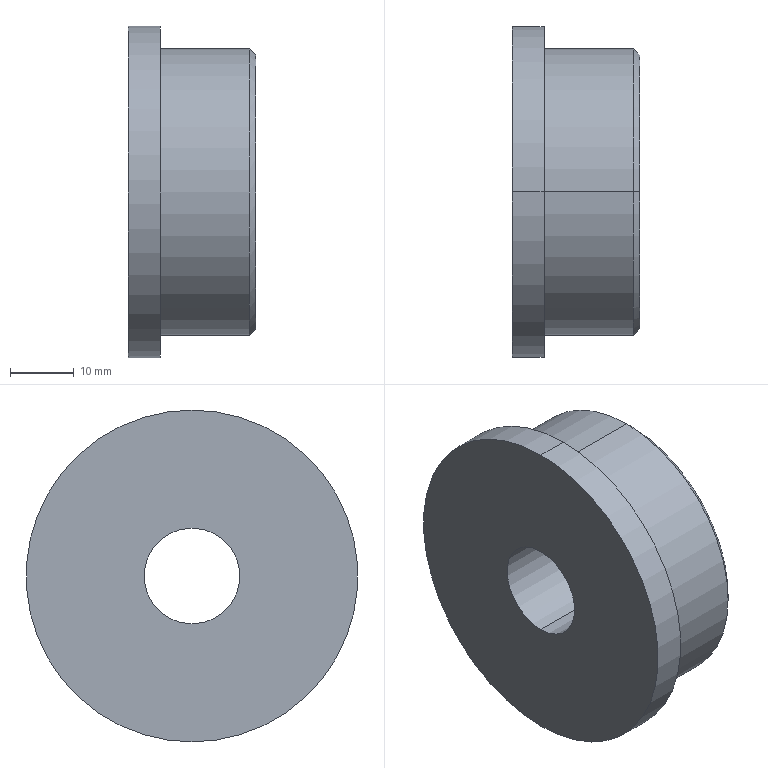Component | SolidWorks | GuideMechanism-1_RollerEndCap02-1 | 1 solid | 11 faces | box 20 x 52 x 52 mm | volume 30871 mm3 | cylinder 6 | plane 3 | cone 2 | commonest cylinder face diameters 52 x2 45 x2 15 x2
build123d program:
from build123d import *

# Parameters (mm, degrees)
CHAMFER1_SIZE = 1


with BuildPart() as part:
    # Sketch1 → Revolve1 (revolve)
    with BuildSketch(Plane.XY, mode=Mode.PRIVATE) as revolve1_sk:
        Polygon((7.5, 0), (7.5, 20), (22.5, 20), (22.5, 5), (26, 5), (26, 0), align=None)
    revolve(revolve1_sk.sketch.rotate(Axis((0, 0, 0), (0, 1, 0)), 90), axis=Axis((0, 0, 0), (0, 1, 0)))

    # Chamfer1
    chamfer1_edges = [part.edges().sort_by_distance(p)[0] for p in [
        (0, 20, 22.5),
    ]]
    chamfer(chamfer1_edges, length=CHAMFER1_SIZE)


solid = part.part

# Placed as in the assembly
solid = solid.moved(Location((-496.772, -352.564, 1209.912), (0, 0, -90)))
STEP:
#1=COLOUR_RGB('',0.7922,0.8196,0.9333);
#2=FILL_AREA_STYLE_COLOUR('',#1);
#3=FILL_AREA_STYLE('',(#2));
#4=SURFACE_STYLE_FILL_AREA(#3);
#5=SURFACE_SIDE_STYLE('',(#4));
#6=SURFACE_STYLE_USAGE(.BOTH.,#5);
#7=PRESENTATION_STYLE_ASSIGNMENT((#6));
#8=CARTESIAN_POINT('',(-18.771,-13.88,48.481));
#9=VERTEX_POINT('',#8);
#10=CARTESIAN_POINT('',(-18.771,-13.88,46.788));
#11=VERTEX_POINT('',#10);
#12=CARTESIAN_POINT('',(-18.771,-13.88,47.634));
#13=DIRECTION('',(1.,0.,0.));
#14=DIRECTION('',(0.,0.,1.));
#15=AXIS2_PLACEMENT_3D('',#12,#13,#14);
#16=CIRCLE('',#15,0.8465);
#17=EDGE_CURVE('',#9,#11,#16,.T.);
#18=ORIENTED_EDGE('',*,*,#17,.F.);
#19=CARTESIAN_POINT('',(-18.81,-13.88,48.52));
#20=VERTEX_POINT('',#19);
#21=CARTESIAN_POINT('',(-18.81,-13.88,48.52));
#22=DIRECTION('',(-0.7071,-0.,0.7071));
#23=VECTOR('',#22,39.37);
#24=LINE('',#21,#23);
#25=EDGE_CURVE('',#9,#20,#24,.T.);
#26=ORIENTED_EDGE('',*,*,#25,.T.);
#27=CARTESIAN_POINT('',(-18.81,-13.88,46.749));
#28=VERTEX_POINT('',#27);
#29=CARTESIAN_POINT('',(-18.81,-13.88,47.634));
#30=DIRECTION('',(-1.,-0.,-0.));
#31=DIRECTION('',(0.,0.,1.));
#32=AXIS2_PLACEMENT_3D('',#29,#30,#31);
#33=CIRCLE('',#32,0.8858);
#34=EDGE_CURVE('',#28,#20,#33,.T.);
#35=ORIENTED_EDGE('',*,*,#34,.F.);
#36=CARTESIAN_POINT('',(-18.81,-13.88,46.749));
#37=DIRECTION('',(-0.7071,0.,-0.7071));
#38=VECTOR('',#37,39.37);
#39=LINE('',#36,#38);
#40=EDGE_CURVE('',#11,#28,#39,.T.);
#41=ORIENTED_EDGE('',*,*,#40,.F.);
#42=EDGE_LOOP('',(#18,#26,#35,#41));
#43=FACE_OUTER_BOUND('',#42,.T.);
#44=CARTESIAN_POINT('',(-18.81,-13.88,47.634));
#45=DIRECTION('',(-1.,-0.,-0.));
#46=DIRECTION('',(0.,0.,-1.));
#47=AXIS2_PLACEMENT_3D('',#44,#45,#46);
#48=CONICAL_SURFACE('',#47,0.8858,0.7854);
#49=ADVANCED_FACE('',(#43),#48,.T.);
#50=CARTESIAN_POINT('',(-19.361,-13.88,46.611));
#51=VERTEX_POINT('',#50);
#52=CARTESIAN_POINT('',(-19.361,-13.88,48.658));
#53=VERTEX_POINT('',#52);
#54=CARTESIAN_POINT('',(-19.361,-13.88,47.634));
#55=DIRECTION('',(-1.,-0.,-0.));
#56=DIRECTION('',(0.,0.,-1.));
#57=AXIS2_PLACEMENT_3D('',#54,#55,#56);
#58=CIRCLE('',#57,1.024);
#59=EDGE_CURVE('',#51,#53,#58,.T.);
#60=ORIENTED_EDGE('',*,*,#59,.T.);
#61=CARTESIAN_POINT('',(-19.558,-13.88,48.658));
#62=VERTEX_POINT('',#61);
#63=CARTESIAN_POINT('',(-19.558,-13.88,48.658));
#64=DIRECTION('',(-1.,-0.,-0.));
#65=VECTOR('',#64,39.37);
#66=LINE('',#63,#65);
#67=EDGE_CURVE('',#53,#62,#66,.T.);
#68=ORIENTED_EDGE('',*,*,#67,.T.);
#69=CARTESIAN_POINT('',(-19.558,-13.88,46.611));
#70=VERTEX_POINT('',#69);
#71=CARTESIAN_POINT('',(-19.558,-13.88,47.634));
#72=DIRECTION('',(-1.,-0.,-0.));
#73=DIRECTION('',(0.,0.,-1.));
#74=AXIS2_PLACEMENT_3D('',#71,#72,#73);
#75=CIRCLE('',#74,1.024);
#76=EDGE_CURVE('',#70,#62,#75,.T.);
#77=ORIENTED_EDGE('',*,*,#76,.F.);
#78=CARTESIAN_POINT('',(-19.558,-13.88,46.611));
#79=DIRECTION('',(-1.,-0.,-0.));
#80=VECTOR('',#79,39.37);
#81=LINE('',#78,#80);
#82=EDGE_CURVE('',#51,#70,#81,.T.);
#83=ORIENTED_EDGE('',*,*,#82,.F.);
#84=EDGE_LOOP('',(#60,#68,#77,#83));
#85=FACE_OUTER_BOUND('',#84,.T.);
#86=CARTESIAN_POINT('',(-19.558,-13.88,47.634));
#87=DIRECTION('',(-1.,-0.,-0.));
#88=DIRECTION('',(0.,0.,-1.));
#89=AXIS2_PLACEMENT_3D('',#86,#87,#88);
#90=CYLINDRICAL_SURFACE('',#89,1.024);
#91=ADVANCED_FACE('',(#85),#90,.T.);
#92=ORIENTED_EDGE('',*,*,#34,.T.);
#93=CARTESIAN_POINT('',(-19.361,-13.88,48.52));
#94=VERTEX_POINT('',#93);
#95=CARTESIAN_POINT('',(-19.558,-13.88,48.52));
#96=DIRECTION('',(-1.,-0.,-0.));
#97=VECTOR('',#96,39.37);
#98=LINE('',#95,#97);
#99=EDGE_CURVE('',#20,#94,#98,.T.);
#100=ORIENTED_EDGE('',*,*,#99,.T.);
#101=CARTESIAN_POINT('',(-19.361,-13.88,46.749));
#102=VERTEX_POINT('',#101);
#103=CARTESIAN_POINT('',(-19.361,-13.88,47.634));
#104=DIRECTION('',(-1.,-0.,-0.));
#105=DIRECTION('',(0.,0.,-1.));
#106=AXIS2_PLACEMENT_3D('',#103,#104,#105);
#107=CIRCLE('',#106,0.8858);
#108=EDGE_CURVE('',#102,#94,#107,.T.);
#109=ORIENTED_EDGE('',*,*,#108,.F.);
#110=CARTESIAN_POINT('',(-19.558,-13.88,46.749));
#111=DIRECTION('',(-1.,-0.,-0.));
#112=VECTOR('',#111,39.37);
#113=LINE('',#110,#112);
#114=EDGE_CURVE('',#28,#102,#113,.T.);
#115=ORIENTED_EDGE('',*,*,#114,.F.);
#116=EDGE_LOOP('',(#92,#100,#109,#115));
#117=FACE_OUTER_BOUND('',#116,.T.);
#118=CARTESIAN_POINT('',(-19.558,-13.88,47.634));
#119=DIRECTION('',(-1.,-0.,-0.));
#120=DIRECTION('',(0.,0.,-1.));
#121=AXIS2_PLACEMENT_3D('',#118,#119,#120);
#122=CYLINDRICAL_SURFACE('',#121,0.8858);
#123=ADVANCED_FACE('',(#117),#122,.T.);
#124=CARTESIAN_POINT('',(-18.771,-13.88,47.93));
#125=VERTEX_POINT('',#124);
#126=CARTESIAN_POINT('',(-18.771,-13.88,47.339));
#127=VERTEX_POINT('',#126);
#128=CARTESIAN_POINT('',(-18.771,-13.88,47.634));
#129=DIRECTION('',(-1.,-0.,-0.));
#130=DIRECTION('',(0.,0.,-1.));
#131=AXIS2_PLACEMENT_3D('',#128,#129,#130);
#132=CIRCLE('',#131,0.2953);
#133=EDGE_CURVE('',#125,#127,#132,.T.);
#134=ORIENTED_EDGE('',*,*,#133,.F.);
#135=CARTESIAN_POINT('',(-19.558,-13.88,47.93));
#136=VERTEX_POINT('',#135);
#137=CARTESIAN_POINT('',(-19.558,-13.88,47.93));
#138=DIRECTION('',(-1.,-0.,-0.));
#139=VECTOR('',#138,39.37);
#140=LINE('',#137,#139);
#141=EDGE_CURVE('',#125,#136,#140,.T.);
#142=ORIENTED_EDGE('',*,*,#141,.T.);
#143=CARTESIAN_POINT('',(-19.558,-13.88,47.339));
#144=VERTEX_POINT('',#143);
#145=CARTESIAN_POINT('',(-19.558,-13.88,47.634));
#146=DIRECTION('',(-1.,-0.,-0.));
#147=DIRECTION('',(0.,0.,-1.));
#148=AXIS2_PLACEMENT_3D('',#145,#146,#147);
#149=CIRCLE('',#148,0.2953);
#150=EDGE_CURVE('',#136,#144,#149,.T.);
#151=ORIENTED_EDGE('',*,*,#150,.T.);
#152=CARTESIAN_POINT('',(-19.558,-13.88,47.339));
#153=DIRECTION('',(-1.,-0.,-0.));
#154=VECTOR('',#153,39.37);
#155=LINE('',#152,#154);
#156=EDGE_CURVE('',#127,#144,#155,.T.);
#157=ORIENTED_EDGE('',*,*,#156,.F.);
#158=EDGE_LOOP('',(#134,#142,#151,#157));
#159=FACE_OUTER_BOUND('',#158,.T.);
#160=CARTESIAN_POINT('',(-19.558,-13.88,47.634));
#161=DIRECTION('',(-1.,-0.,-0.));
#162=DIRECTION('',(0.,0.,-1.));
#163=AXIS2_PLACEMENT_3D('',#160,#161,#162);
#164=CYLINDRICAL_SURFACE('',#163,0.2953);
#165=ADVANCED_FACE('',(#159),#164,.F.);
#166=ORIENTED_EDGE('',*,*,#76,.T.);
#167=CARTESIAN_POINT('',(-19.558,-13.88,47.634));
#168=DIRECTION('',(-1.,-0.,-0.));
#169=DIRECTION('',(0.,0.,-1.));
#170=AXIS2_PLACEMENT_3D('',#167,#168,#169);
#171=CIRCLE('',#170,1.024);
#172=EDGE_CURVE('',#62,#70,#171,.T.);
#173=ORIENTED_EDGE('',*,*,#172,.T.);
#174=EDGE_LOOP('',(#166,#173));
#175=FACE_OUTER_BOUND('',#174,.T.);
#176=CARTESIAN_POINT('',(-19.558,-13.88,47.634));
#177=DIRECTION('',(-1.,-0.,-0.));
#178=DIRECTION('',(0.,0.,-1.));
#179=AXIS2_PLACEMENT_3D('',#176,#177,#178);
#180=CIRCLE('',#179,0.2953);
#181=EDGE_CURVE('',#144,#136,#180,.T.);
#182=ORIENTED_EDGE('',*,*,#181,.F.);
#183=ORIENTED_EDGE('',*,*,#150,.F.);
#184=EDGE_LOOP('',(#182,#183));
#185=FACE_BOUND('',#184,.T.);
#186=CARTESIAN_POINT('',(-19.558,-14.904,47.634));
#187=DIRECTION('',(-1.,-0.,-0.));
#188=DIRECTION('',(0.,0.,-1.));
#189=AXIS2_PLACEMENT_3D('',#186,#187,#188);
#190=PLANE('',#189);
#191=ADVANCED_FACE('',(#175,#185),#190,.T.);
#192=ORIENTED_EDGE('',*,*,#141,.F.);
#193=CARTESIAN_POINT('',(-18.771,-13.88,47.634));
#194=DIRECTION('',(-1.,-0.,-0.));
#195=DIRECTION('',(0.,0.,-1.));
#196=AXIS2_PLACEMENT_3D('',#193,#194,#195);
#197=CIRCLE('',#196,0.2953);
#198=EDGE_CURVE('',#127,#125,#197,.T.);
#199=ORIENTED_EDGE('',*,*,#198,.F.);
#200=ORIENTED_EDGE('',*,*,#156,.T.);
#201=ORIENTED_EDGE('',*,*,#181,.T.);
#202=EDGE_LOOP('',(#192,#199,#200,#201));
#203=FACE_OUTER_BOUND('',#202,.T.);
#204=CARTESIAN_POINT('',(-19.558,-13.88,47.634));
#205=DIRECTION('',(-1.,-0.,-0.));
#206=DIRECTION('',(0.,0.,-1.));
#207=AXIS2_PLACEMENT_3D('',#204,#205,#206);
#208=CYLINDRICAL_SURFACE('',#207,0.2953);
#209=ADVANCED_FACE('',(#203),#208,.F.);
#210=CARTESIAN_POINT('',(-18.771,-13.88,47.634));
#211=DIRECTION('',(1.,0.,0.));
#212=DIRECTION('',(0.,0.,1.));
#213=AXIS2_PLACEMENT_3D('',#210,#211,#212);
#214=CIRCLE('',#213,0.8465);
#215=EDGE_CURVE('',#11,#9,#214,.T.);
#216=ORIENTED_EDGE('',*,*,#215,.T.);
#217=ORIENTED_EDGE('',*,*,#17,.T.);
#218=EDGE_LOOP('',(#216,#217));
#219=FACE_OUTER_BOUND('',#218,.T.);
#220=ORIENTED_EDGE('',*,*,#198,.T.);
#221=ORIENTED_EDGE('',*,*,#133,.T.);
#222=EDGE_LOOP('',(#220,#221));
#223=FACE_BOUND('',#222,.T.);
#224=CARTESIAN_POINT('',(-18.771,-14.176,47.634));
#225=DIRECTION('',(1.,0.,0.));
#226=DIRECTION('',(-0.,-0.,1.));
#227=AXIS2_PLACEMENT_3D('',#224,#225,#226);
#228=PLANE('',#227);
#229=ADVANCED_FACE('',(#219,#223),#228,.T.);
#230=ORIENTED_EDGE('',*,*,#99,.F.);
#231=CARTESIAN_POINT('',(-18.81,-13.88,47.634));
#232=DIRECTION('',(-1.,-0.,-0.));
#233=DIRECTION('',(0.,0.,1.));
#234=AXIS2_PLACEMENT_3D('',#231,#232,#233);
#235=CIRCLE('',#234,0.8858);
#236=EDGE_CURVE('',#20,#28,#235,.T.);
#237=ORIENTED_EDGE('',*,*,#236,.T.);
#238=ORIENTED_EDGE('',*,*,#114,.T.);
#239=CARTESIAN_POINT('',(-19.361,-13.88,47.634));
#240=DIRECTION('',(-1.,-0.,-0.));
#241=DIRECTION('',(0.,0.,-1.));
#242=AXIS2_PLACEMENT_3D('',#239,#240,#241);
#243=CIRCLE('',#242,0.8858);
#244=EDGE_CURVE('',#94,#102,#243,.T.);
#245=ORIENTED_EDGE('',*,*,#244,.F.);
#246=EDGE_LOOP('',(#230,#237,#238,#245));
#247=FACE_OUTER_BOUND('',#246,.T.);
#248=CARTESIAN_POINT('',(-19.558,-13.88,47.634));
#249=DIRECTION('',(-1.,-0.,-0.));
#250=DIRECTION('',(0.,0.,-1.));
#251=AXIS2_PLACEMENT_3D('',#248,#249,#250);
#252=CYLINDRICAL_SURFACE('',#251,0.8858);
#253=ADVANCED_FACE('',(#247),#252,.T.);
#254=ORIENTED_EDGE('',*,*,#108,.T.);
#255=ORIENTED_EDGE('',*,*,#244,.T.);
#256=EDGE_LOOP('',(#254,#255));
#257=FACE_BOUND('',#256,.T.);
#258=ORIENTED_EDGE('',*,*,#59,.F.);
#259=CARTESIAN_POINT('',(-19.361,-13.88,47.634));
#260=DIRECTION('',(-1.,-0.,-0.));
#261=DIRECTION('',(0.,0.,-1.));
#262=AXIS2_PLACEMENT_3D('',#259,#260,#261);
#263=CIRCLE('',#262,1.024);
#264=EDGE_CURVE('',#53,#51,#263,.T.);
#265=ORIENTED_EDGE('',*,*,#264,.F.);
#266=EDGE_LOOP('',(#258,#265));
#267=FACE_OUTER_BOUND('',#266,.T.);
#268=CARTESIAN_POINT('',(-19.361,-14.766,47.634));
#269=DIRECTION('',(1.,0.,0.));
#270=DIRECTION('',(-0.,-0.,1.));
#271=AXIS2_PLACEMENT_3D('',#268,#269,#270);
#272=PLANE('',#271);
#273=ADVANCED_FACE('',(#257,#267),#272,.T.);
#274=ORIENTED_EDGE('',*,*,#67,.F.);
#275=ORIENTED_EDGE('',*,*,#264,.T.);
#276=ORIENTED_EDGE('',*,*,#82,.T.);
#277=ORIENTED_EDGE('',*,*,#172,.F.);
#278=EDGE_LOOP('',(#274,#275,#276,#277));
#279=FACE_OUTER_BOUND('',#278,.T.);
#280=CARTESIAN_POINT('',(-19.558,-13.88,47.634));
#281=DIRECTION('',(-1.,-0.,-0.));
#282=DIRECTION('',(0.,0.,-1.));
#283=AXIS2_PLACEMENT_3D('',#280,#281,#282);
#284=CYLINDRICAL_SURFACE('',#283,1.024);
#285=ADVANCED_FACE('',(#279),#284,.T.);
#286=ORIENTED_EDGE('',*,*,#25,.F.);
#287=ORIENTED_EDGE('',*,*,#215,.F.);
#288=ORIENTED_EDGE('',*,*,#40,.T.);
#289=ORIENTED_EDGE('',*,*,#236,.F.);
#290=EDGE_LOOP('',(#286,#287,#288,#289));
#291=FACE_OUTER_BOUND('',#290,.T.);
#292=CARTESIAN_POINT('',(-18.81,-13.88,47.634));
#293=DIRECTION('',(-1.,-0.,-0.));
#294=DIRECTION('',(0.,0.,-1.));
#295=AXIS2_PLACEMENT_3D('',#292,#293,#294);
#296=CONICAL_SURFACE('',#295,0.8858,0.7854);
#297=ADVANCED_FACE('',(#291),#296,.T.);
#298=CLOSED_SHELL('',(#49,#91,#123,#165,#191,#209,#229,#253,#273,#285,#297));
#299=MANIFOLD_SOLID_BREP('',#298);
#300=STYLED_ITEM('',(#7),#299);
#301=(LENGTH_UNIT()NAMED_UNIT(*)SI_UNIT($,.METRE.));
#302=LENGTH_MEASURE_WITH_UNIT(LENGTH_MEASURE(0.0254),#301);
#303=DIMENSIONAL_EXPONENTS(1.,0.,0.,0.,0.,0.,0.);
#304=(CONVERSION_BASED_UNIT('',#302)LENGTH_UNIT()NAMED_UNIT(#303));
#305=UNCERTAINTY_MEASURE_WITH_UNIT(LENGTH_MEASURE(0.00001),#304,'','');
#306=(NAMED_UNIT(*)PLANE_ANGLE_UNIT()SI_UNIT($,.RADIAN.));
#307=(NAMED_UNIT(*)SI_UNIT($,.STERADIAN.)SOLID_ANGLE_UNIT());
#308=(GEOMETRIC_REPRESENTATION_CONTEXT(3)GLOBAL_UNCERTAINTY_ASSIGNED_CONTEXT((#305))GLOBAL_UNIT_ASSIGNED_CONTEXT((#304,#306,#307))REPRESENTATION_CONTEXT('',''));
#309=MECHANICAL_DESIGN_GEOMETRIC_PRESENTATION_REPRESENTATION('',(#300),#308);
#310=PRESENTATION_LAYER_ASSIGNMENT('','',(#300));
#311=CARTESIAN_POINT('',(0.,0.,0.));
#312=DIRECTION('',(0.,0.,1.));
#313=DIRECTION('',(1.,0.,0.));
#314=AXIS2_PLACEMENT_3D('',#311,#312,#313);
#315=(LENGTH_UNIT()NAMED_UNIT(*)SI_UNIT($,.METRE.));
#316=LENGTH_MEASURE_WITH_UNIT(LENGTH_MEASURE(0.0254),#315);
#317=DIMENSIONAL_EXPONENTS(1.,0.,0.,0.,0.,0.,0.);
#318=(CONVERSION_BASED_UNIT('',#316)LENGTH_UNIT()NAMED_UNIT(#317));
#319=UNCERTAINTY_MEASURE_WITH_UNIT(LENGTH_MEASURE(0.00001),#318,'','');
#320=(NAMED_UNIT(*)PLANE_ANGLE_UNIT()SI_UNIT($,.RADIAN.));
#321=(NAMED_UNIT(*)SI_UNIT($,.STERADIAN.)SOLID_ANGLE_UNIT());
#322=(GEOMETRIC_REPRESENTATION_CONTEXT(3)GLOBAL_UNCERTAINTY_ASSIGNED_CONTEXT((#319))GLOBAL_UNIT_ASSIGNED_CONTEXT((#318,#320,#321))REPRESENTATION_CONTEXT('',''));
#323=ADVANCED_BREP_SHAPE_REPRESENTATION('',(#299,#314),#322);